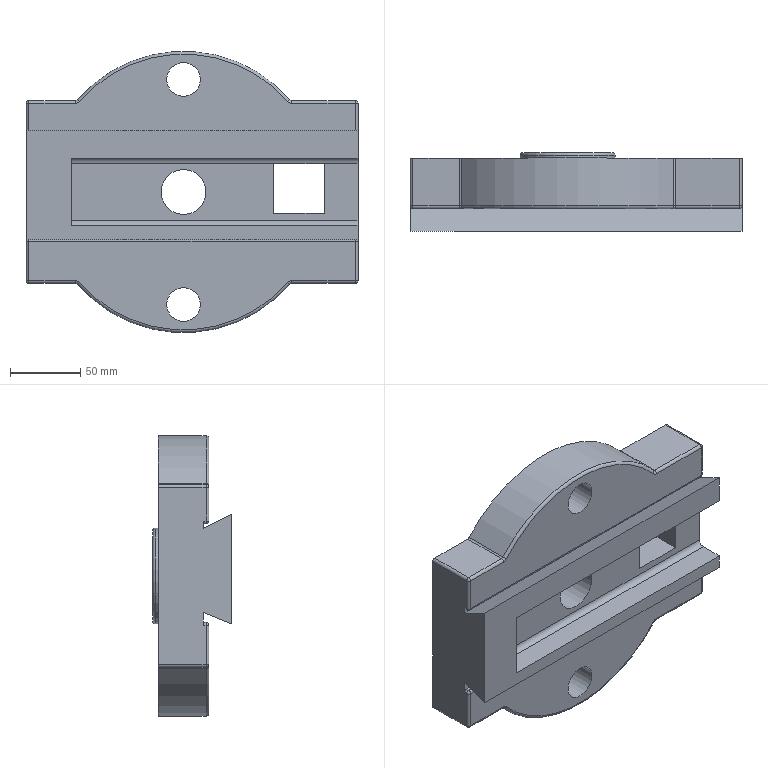Component | NX | TOOL_HOLDER_BASE | 1 solid | 73 faces | volume 1334993 mm3 | cylinder 30 | plane 26 | torus 9 | sphere 8 | commonest cylinder face diameters 4 x22 200 x2 24 x2 8 x2 68 x1 32 x1